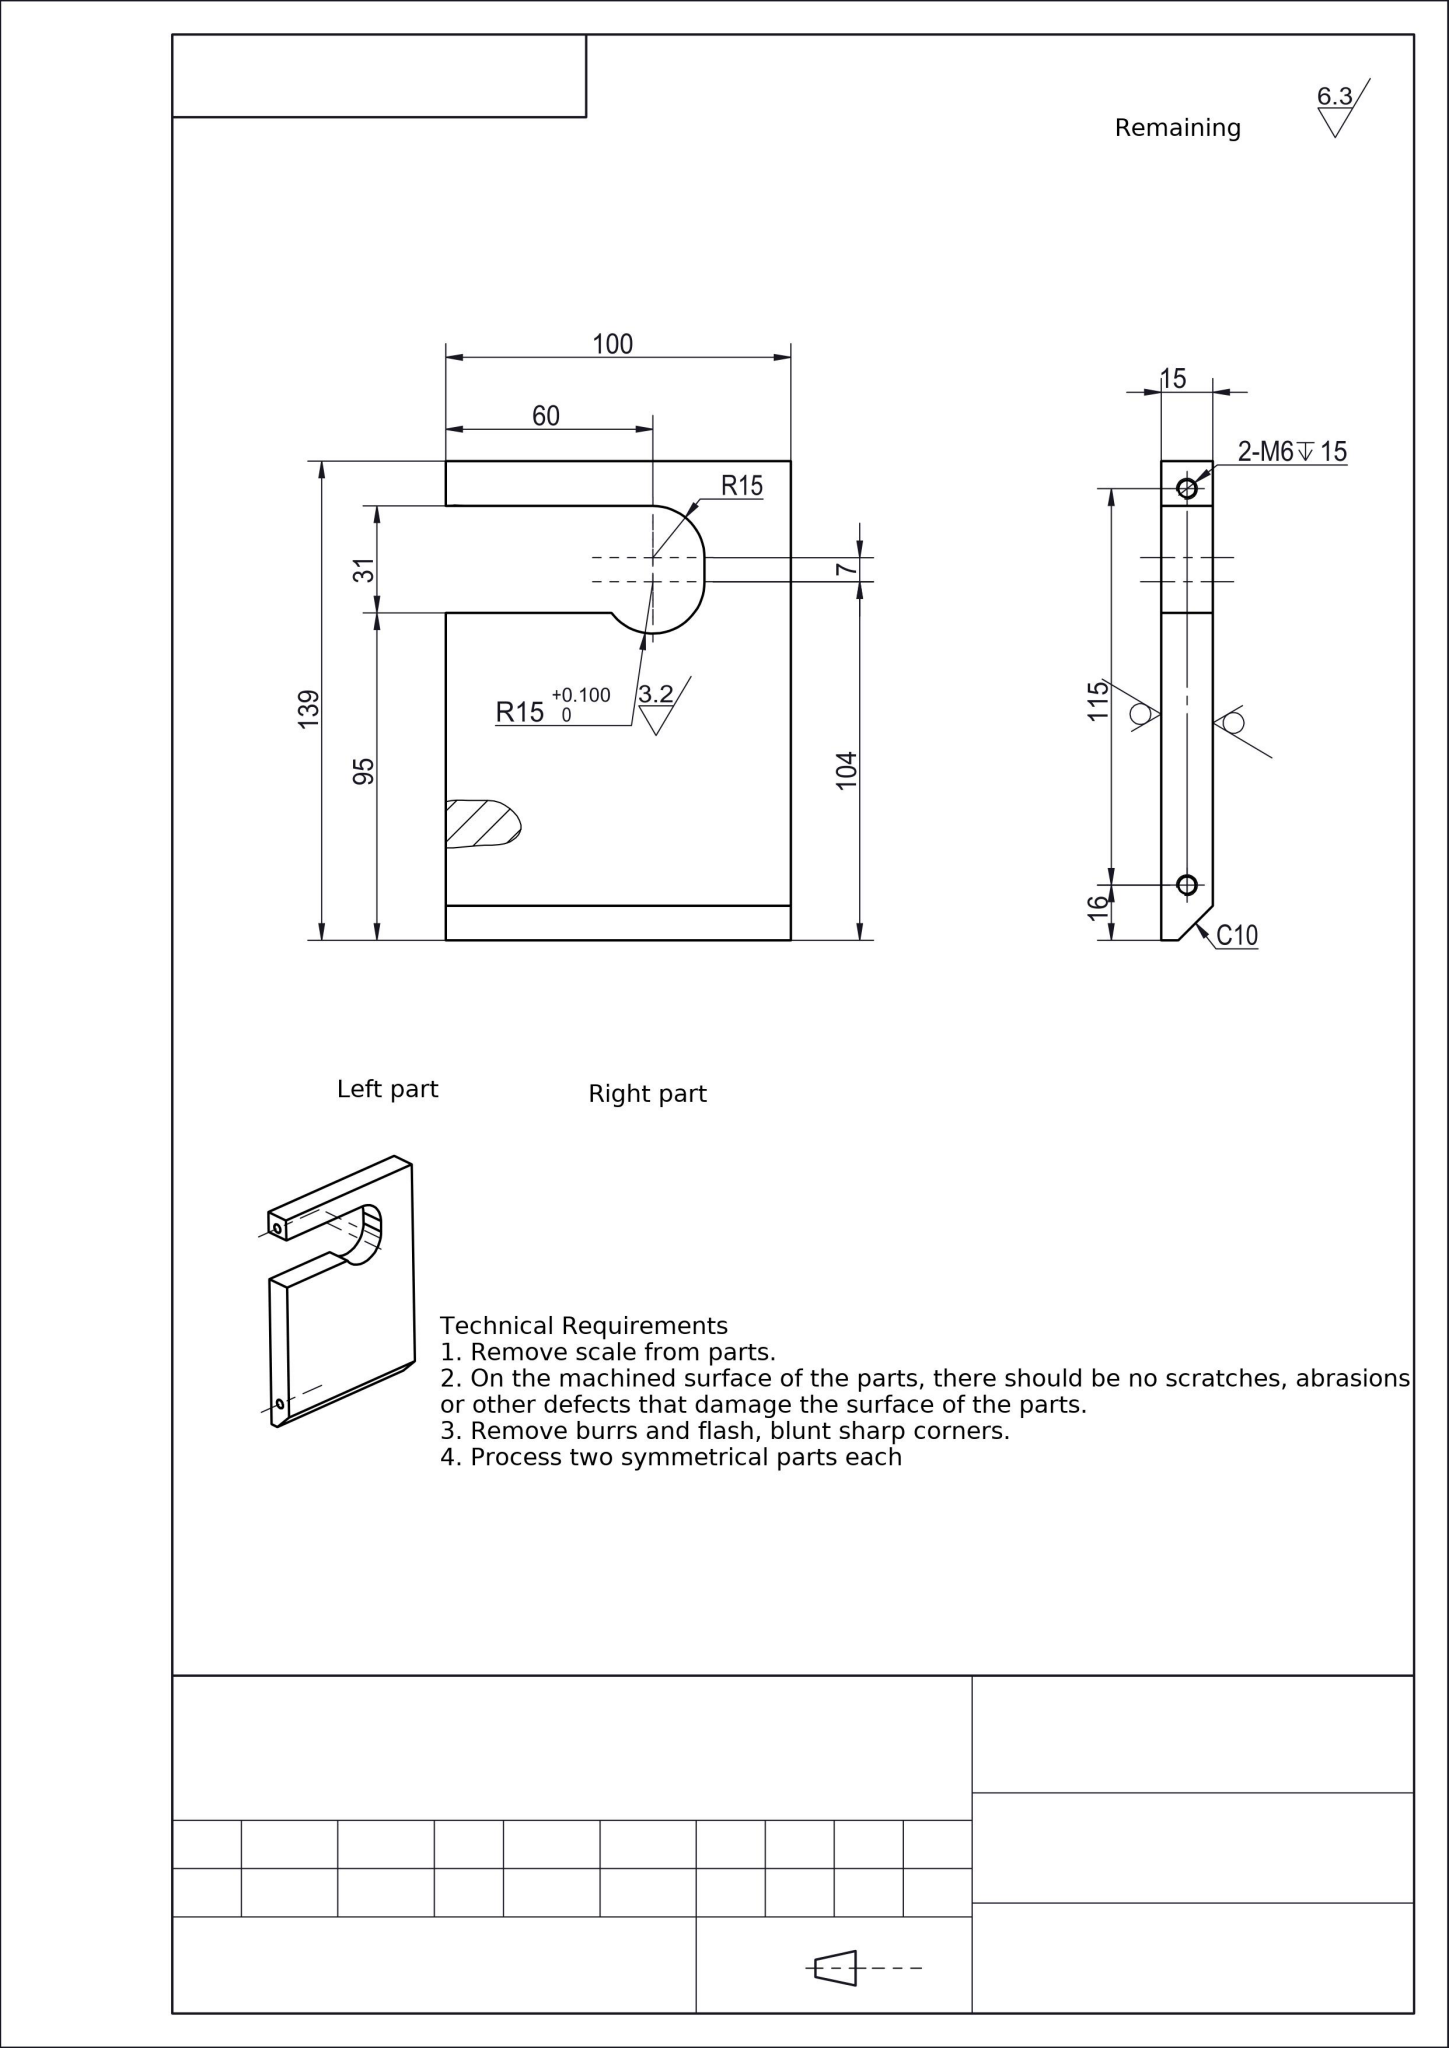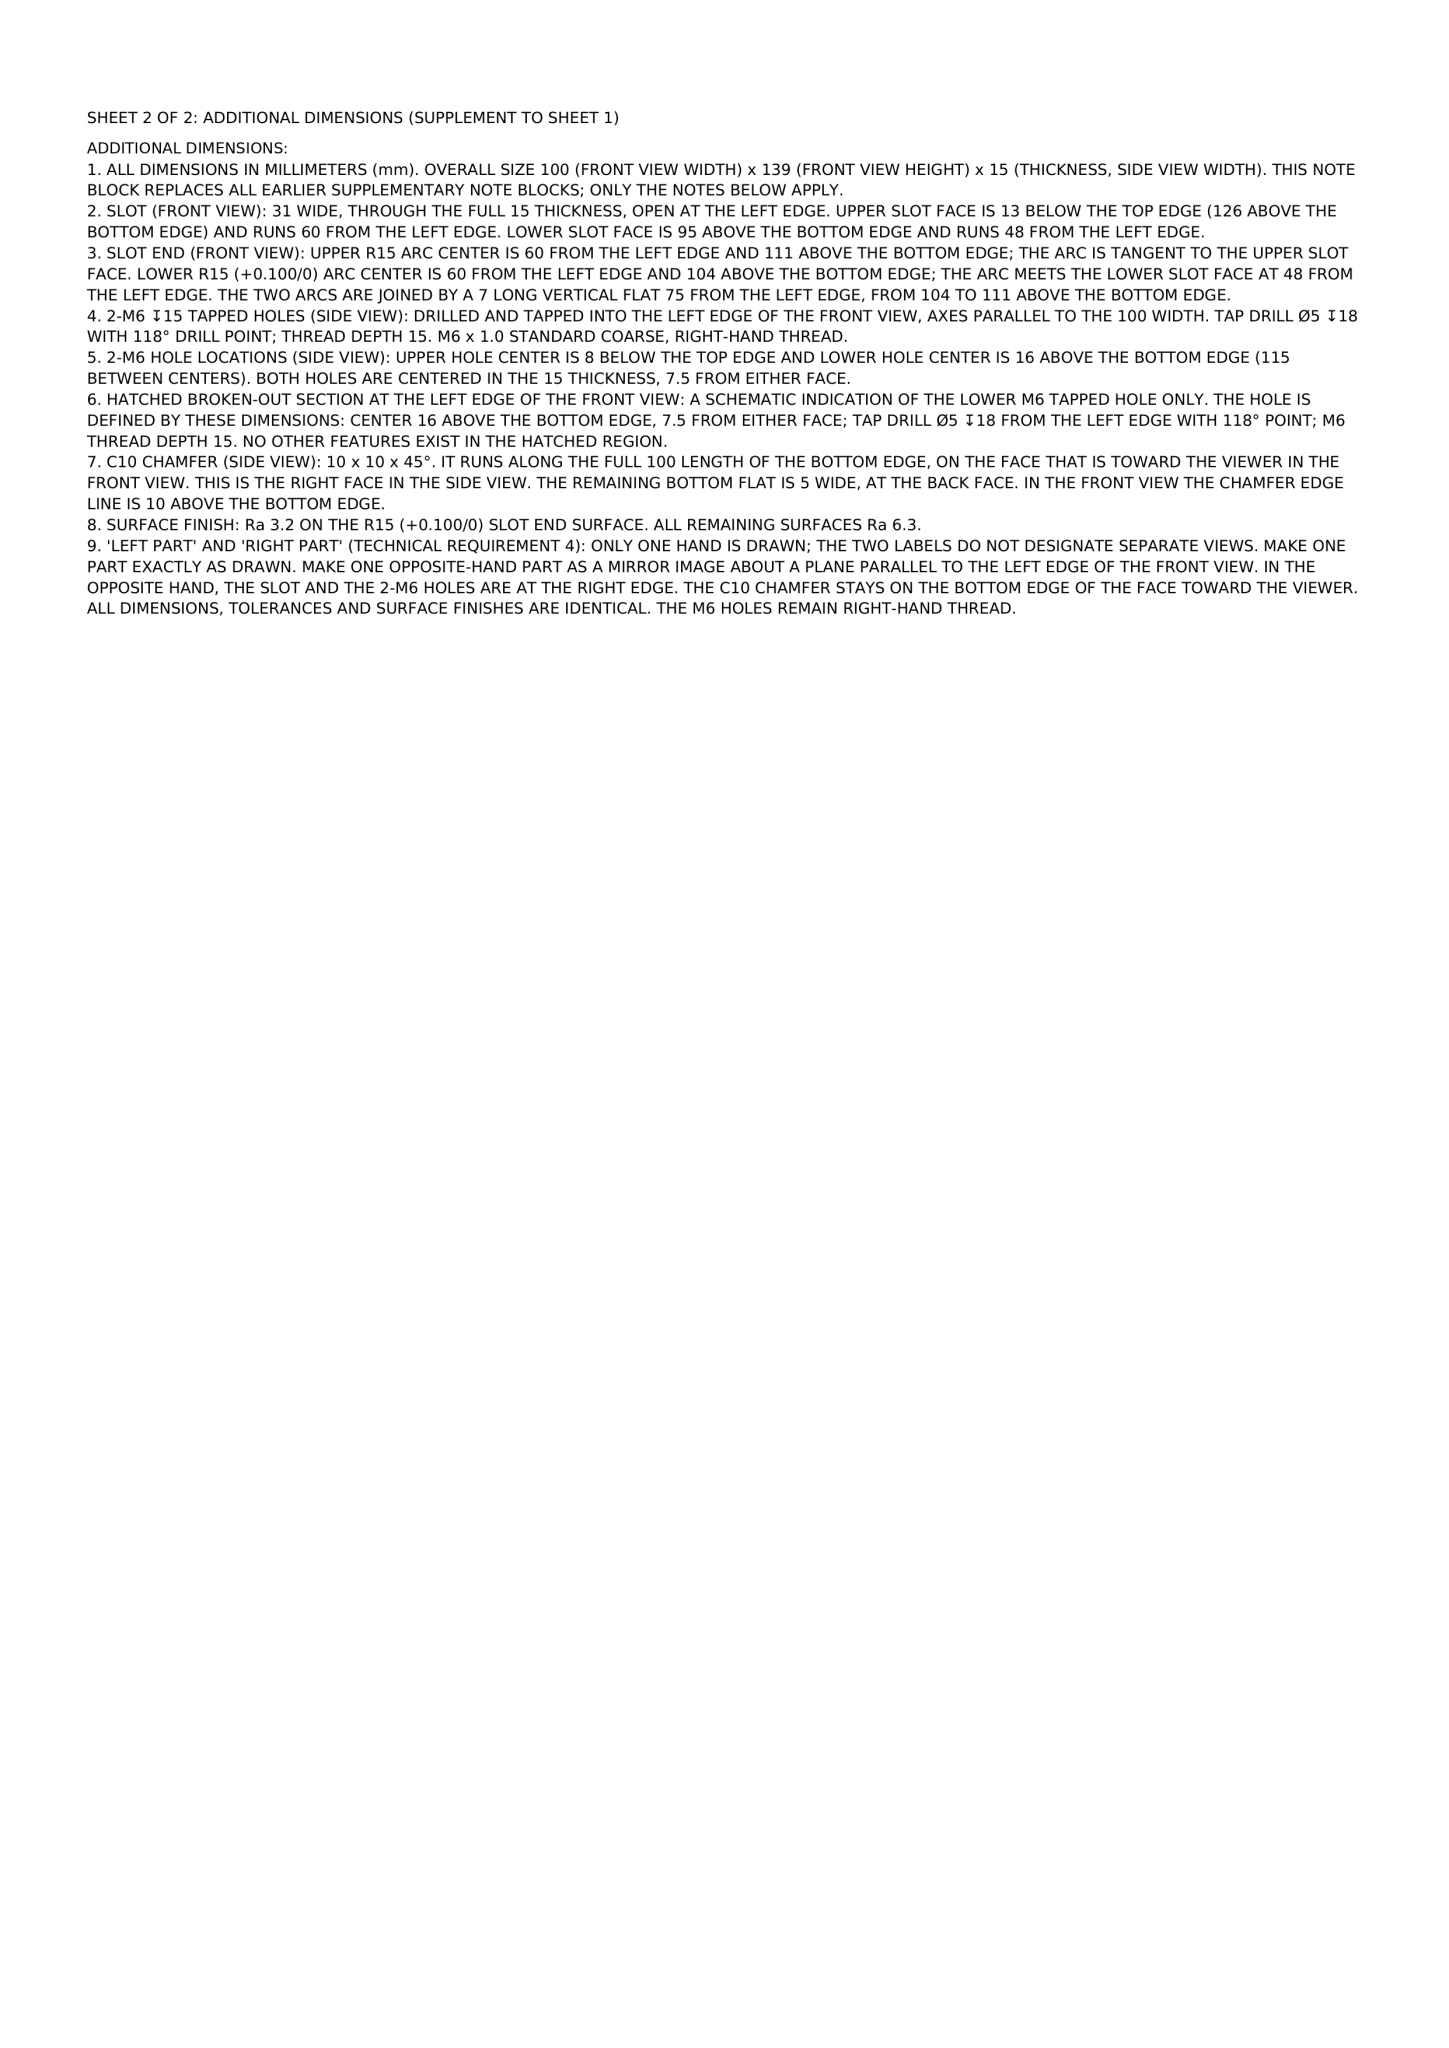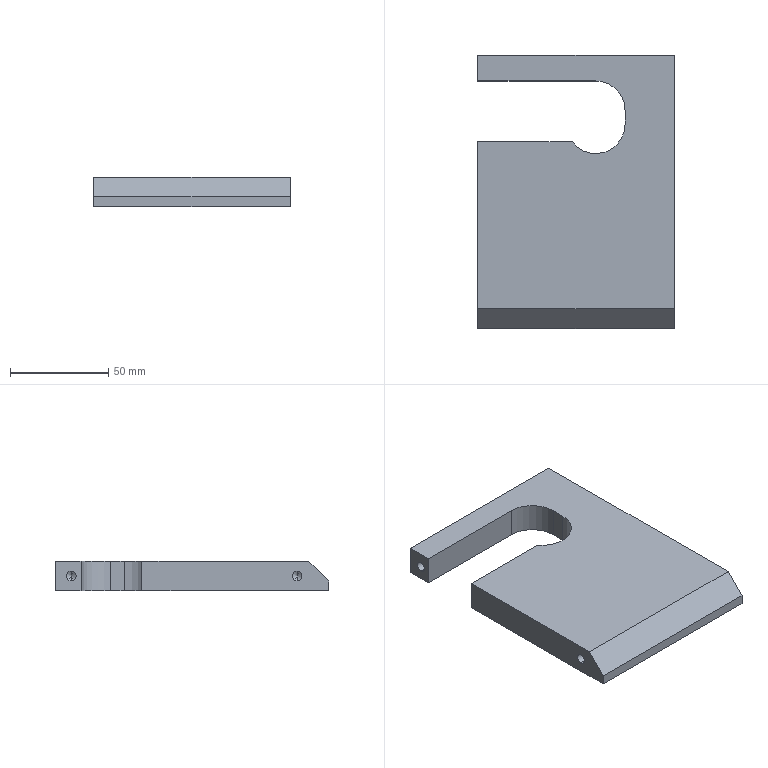Part | NX | mm | 1 solid | 21 faces | box 100 x 139 x 15 mm | volume 167242 mm3 | plane 11 | cylinder 6 | cone 4 | commonest cylinder face diameters 5 x4 30 x2
STEP:
#1=COLOUR_RGB('',0.7529,0.7529,0.7529);
#2=FILL_AREA_STYLE_COLOUR('',#1);
#3=FILL_AREA_STYLE('',(#2));
#4=SURFACE_STYLE_FILL_AREA(#3);
#5=SURFACE_SIDE_STYLE('',(#4));
#6=SURFACE_STYLE_USAGE(.BOTH.,#5);
#7=PRESENTATION_STYLE_ASSIGNMENT((#6));
#8=CARTESIAN_POINT('',(-32.,61.5,5.));
#9=VERTEX_POINT('',#8);
#10=CARTESIAN_POINT('',(-32.,61.5,10.));
#11=VERTEX_POINT('',#10);
#12=CARTESIAN_POINT('',(-32.,61.5,7.5));
#13=DIRECTION('',(-1.,-0.,0.));
#14=DIRECTION('',(0.,0.,1.));
#15=AXIS2_PLACEMENT_3D('',#12,#13,#14);
#16=CIRCLE('',#15,2.5);
#17=EDGE_CURVE('',#9,#11,#16,.T.);
#18=ORIENTED_EDGE('',*,*,#17,.F.);
#19=CARTESIAN_POINT('',(-50.,61.5,5.));
#20=VERTEX_POINT('',#19);
#21=CARTESIAN_POINT('',(-50.,61.5,5.));
#22=DIRECTION('',(-1.,-0.,0.));
#23=VECTOR('',#22,1000.);
#24=LINE('',#21,#23);
#25=EDGE_CURVE('',#9,#20,#24,.T.);
#26=ORIENTED_EDGE('',*,*,#25,.T.);
#27=CARTESIAN_POINT('',(-50.,61.5,10.));
#28=VERTEX_POINT('',#27);
#29=CARTESIAN_POINT('',(-50.,61.5,7.5));
#30=DIRECTION('',(-1.,-0.,0.));
#31=DIRECTION('',(0.,0.,1.));
#32=AXIS2_PLACEMENT_3D('',#29,#30,#31);
#33=CIRCLE('',#32,2.5);
#34=EDGE_CURVE('',#20,#28,#33,.T.);
#35=ORIENTED_EDGE('',*,*,#34,.T.);
#36=CARTESIAN_POINT('',(-50.,61.5,10.));
#37=DIRECTION('',(-1.,-0.,0.));
#38=VECTOR('',#37,1000.);
#39=LINE('',#36,#38);
#40=EDGE_CURVE('',#11,#28,#39,.T.);
#41=ORIENTED_EDGE('',*,*,#40,.F.);
#42=EDGE_LOOP('',(#18,#26,#35,#41));
#43=FACE_OUTER_BOUND('',#42,.T.);
#44=CARTESIAN_POINT('',(-50.,61.5,7.5));
#45=DIRECTION('',(-1.,-0.,0.));
#46=DIRECTION('',(0.,0.,1.));
#47=AXIS2_PLACEMENT_3D('',#44,#45,#46);
#48=CYLINDRICAL_SURFACE('',#47,2.5);
#49=ADVANCED_FACE('',(#43),#48,.F.);
#50=STYLED_ITEM('',(#7),#49);
#51=(LENGTH_UNIT()NAMED_UNIT(*)SI_UNIT(.MILLI.,.METRE.));
#52=UNCERTAINTY_MEASURE_WITH_UNIT(LENGTH_MEASURE(0.00001),#51,'','');
#53=(NAMED_UNIT(*)PLANE_ANGLE_UNIT()SI_UNIT($,.RADIAN.));
#54=(NAMED_UNIT(*)SI_UNIT($,.STERADIAN.)SOLID_ANGLE_UNIT());
#55=(GEOMETRIC_REPRESENTATION_CONTEXT(3)GLOBAL_UNCERTAINTY_ASSIGNED_CONTEXT((#52))GLOBAL_UNIT_ASSIGNED_CONTEXT((#51,#53,#54))REPRESENTATION_CONTEXT('',''));
#56=MECHANICAL_DESIGN_GEOMETRIC_PRESENTATION_REPRESENTATION('',(#50),#55);
#57=COLOUR_RGB('',1.,1.,1.);
#58=FILL_AREA_STYLE_COLOUR('',#57);
#59=FILL_AREA_STYLE('',(#58));
#60=SURFACE_STYLE_FILL_AREA(#59);
#61=SURFACE_SIDE_STYLE('',(#60));
#62=SURFACE_STYLE_USAGE(.BOTH.,#61);
#63=PRESENTATION_STYLE_ASSIGNMENT((#62));
#64=CARTESIAN_POINT('',(-30.498,61.5,7.5));
#65=VERTEX_POINT('',#64);
#66=CARTESIAN_POINT('',(-32.,61.5,10.));
#67=DIRECTION('',(-0.515,-0.,0.8572));
#68=VECTOR('',#67,1000.);
#69=LINE('',#66,#68);
#70=EDGE_CURVE('',#65,#11,#69,.T.);
#71=ORIENTED_EDGE('',*,*,#70,.F.);
#72=CARTESIAN_POINT('',(-32.,61.5,5.));
#73=DIRECTION('',(-0.515,0.,-0.8572));
#74=VECTOR('',#73,1000.);
#75=LINE('',#72,#74);
#76=EDGE_CURVE('',#65,#9,#75,.T.);
#77=ORIENTED_EDGE('',*,*,#76,.T.);
#78=ORIENTED_EDGE('',*,*,#17,.T.);
#79=EDGE_LOOP('',(#71,#77,#78));
#80=FACE_OUTER_BOUND('',#79,.T.);
#81=CARTESIAN_POINT('',(-32.,61.5,7.5));
#82=DIRECTION('',(-1.,-0.,0.));
#83=DIRECTION('',(0.,0.,1.));
#84=AXIS2_PLACEMENT_3D('',#81,#82,#83);
#85=CONICAL_SURFACE('',#84,2.5,1.03);
#86=ADVANCED_FACE('',(#80),#85,.F.);
#87=CARTESIAN_POINT('',(-32.,-53.5,5.));
#88=VERTEX_POINT('',#87);
#89=CARTESIAN_POINT('',(-32.,-53.5,10.));
#90=VERTEX_POINT('',#89);
#91=CARTESIAN_POINT('',(-32.,-53.5,7.5));
#92=DIRECTION('',(-1.,-0.,0.));
#93=DIRECTION('',(0.,0.,1.));
#94=AXIS2_PLACEMENT_3D('',#91,#92,#93);
#95=CIRCLE('',#94,2.5);
#96=EDGE_CURVE('',#88,#90,#95,.T.);
#97=ORIENTED_EDGE('',*,*,#96,.F.);
#98=CARTESIAN_POINT('',(-50.,-53.5,5.));
#99=VERTEX_POINT('',#98);
#100=CARTESIAN_POINT('',(-50.,-53.5,5.));
#101=DIRECTION('',(-1.,-0.,0.));
#102=VECTOR('',#101,1000.);
#103=LINE('',#100,#102);
#104=EDGE_CURVE('',#88,#99,#103,.T.);
#105=ORIENTED_EDGE('',*,*,#104,.T.);
#106=CARTESIAN_POINT('',(-50.,-53.5,10.));
#107=VERTEX_POINT('',#106);
#108=CARTESIAN_POINT('',(-50.,-53.5,7.5));
#109=DIRECTION('',(-1.,-0.,0.));
#110=DIRECTION('',(0.,0.,1.));
#111=AXIS2_PLACEMENT_3D('',#108,#109,#110);
#112=CIRCLE('',#111,2.5);
#113=EDGE_CURVE('',#99,#107,#112,.T.);
#114=ORIENTED_EDGE('',*,*,#113,.T.);
#115=CARTESIAN_POINT('',(-50.,-53.5,10.));
#116=DIRECTION('',(-1.,-0.,0.));
#117=VECTOR('',#116,1000.);
#118=LINE('',#115,#117);
#119=EDGE_CURVE('',#90,#107,#118,.T.);
#120=ORIENTED_EDGE('',*,*,#119,.F.);
#121=EDGE_LOOP('',(#97,#105,#114,#120));
#122=FACE_OUTER_BOUND('',#121,.T.);
#123=CARTESIAN_POINT('',(-50.,-53.5,7.5));
#124=DIRECTION('',(-1.,-0.,0.));
#125=DIRECTION('',(0.,0.,1.));
#126=AXIS2_PLACEMENT_3D('',#123,#124,#125);
#127=CYLINDRICAL_SURFACE('',#126,2.5);
#128=ADVANCED_FACE('',(#122),#127,.F.);
#129=CARTESIAN_POINT('',(-30.498,-53.5,7.5));
#130=VERTEX_POINT('',#129);
#131=CARTESIAN_POINT('',(-32.,-53.5,10.));
#132=DIRECTION('',(-0.515,-0.,0.8572));
#133=VECTOR('',#132,1000.);
#134=LINE('',#131,#133);
#135=EDGE_CURVE('',#130,#90,#134,.T.);
#136=ORIENTED_EDGE('',*,*,#135,.F.);
#137=CARTESIAN_POINT('',(-32.,-53.5,5.));
#138=DIRECTION('',(-0.515,0.,-0.8572));
#139=VECTOR('',#138,1000.);
#140=LINE('',#137,#139);
#141=EDGE_CURVE('',#130,#88,#140,.T.);
#142=ORIENTED_EDGE('',*,*,#141,.T.);
#143=ORIENTED_EDGE('',*,*,#96,.T.);
#144=EDGE_LOOP('',(#136,#142,#143));
#145=FACE_OUTER_BOUND('',#144,.T.);
#146=CARTESIAN_POINT('',(-32.,-53.5,7.5));
#147=DIRECTION('',(-1.,-0.,0.));
#148=DIRECTION('',(0.,0.,1.));
#149=AXIS2_PLACEMENT_3D('',#146,#147,#148);
#150=CONICAL_SURFACE('',#149,2.5,1.03);
#151=ADVANCED_FACE('',(#145),#150,.F.);
#152=CARTESIAN_POINT('',(-50.,25.5,15.));
#153=VERTEX_POINT('',#152);
#154=CARTESIAN_POINT('',(-50.,-59.5,15.));
#155=VERTEX_POINT('',#154);
#156=CARTESIAN_POINT('',(-50.,69.5,15.));
#157=DIRECTION('',(0.,-1.,0.));
#158=VECTOR('',#157,1000.);
#159=LINE('',#156,#158);
#160=EDGE_CURVE('',#153,#155,#159,.T.);
#161=ORIENTED_EDGE('',*,*,#160,.T.);
#162=CARTESIAN_POINT('',(50.,-59.5,15.));
#163=VERTEX_POINT('',#162);
#164=CARTESIAN_POINT('',(50.,-59.5,15.));
#165=DIRECTION('',(1.,0.,-0.));
#166=VECTOR('',#165,1000.);
#167=LINE('',#164,#166);
#168=EDGE_CURVE('',#155,#163,#167,.T.);
#169=ORIENTED_EDGE('',*,*,#168,.T.);
#170=CARTESIAN_POINT('',(50.,69.5,15.));
#171=VERTEX_POINT('',#170);
#172=CARTESIAN_POINT('',(50.,69.5,15.));
#173=DIRECTION('',(0.,1.,-0.));
#174=VECTOR('',#173,1000.);
#175=LINE('',#172,#174);
#176=EDGE_CURVE('',#163,#171,#175,.T.);
#177=ORIENTED_EDGE('',*,*,#176,.T.);
#178=CARTESIAN_POINT('',(-50.,69.5,15.));
#179=VERTEX_POINT('',#178);
#180=CARTESIAN_POINT('',(-50.,69.5,15.));
#181=DIRECTION('',(-1.,-0.,0.));
#182=VECTOR('',#181,1000.);
#183=LINE('',#180,#182);
#184=EDGE_CURVE('',#171,#179,#183,.T.);
#185=ORIENTED_EDGE('',*,*,#184,.T.);
#186=CARTESIAN_POINT('',(-50.,56.5,15.));
#187=VERTEX_POINT('',#186);
#188=CARTESIAN_POINT('',(-50.,69.5,15.));
#189=DIRECTION('',(0.,-1.,0.));
#190=VECTOR('',#189,1000.);
#191=LINE('',#188,#190);
#192=EDGE_CURVE('',#179,#187,#191,.T.);
#193=ORIENTED_EDGE('',*,*,#192,.T.);
#194=CARTESIAN_POINT('',(10.,56.5,15.));
#195=VERTEX_POINT('',#194);
#196=CARTESIAN_POINT('',(-112.137,56.5,15.));
#197=DIRECTION('',(-1.,-0.,0.));
#198=VECTOR('',#197,1000.);
#199=LINE('',#196,#198);
#200=EDGE_CURVE('',#195,#187,#199,.T.);
#201=ORIENTED_EDGE('',*,*,#200,.F.);
#202=CARTESIAN_POINT('',(25.,41.5,15.));
#203=VERTEX_POINT('',#202);
#204=CARTESIAN_POINT('',(10.,41.5,15.));
#205=DIRECTION('',(-0.,-0.,1.));
#206=DIRECTION('',(1.,0.,-0.));
#207=AXIS2_PLACEMENT_3D('',#204,#205,#206);
#208=CIRCLE('',#207,15.);
#209=EDGE_CURVE('',#203,#195,#208,.T.);
#210=ORIENTED_EDGE('',*,*,#209,.F.);
#211=CARTESIAN_POINT('',(25.,34.5,15.));
#212=VERTEX_POINT('',#211);
#213=CARTESIAN_POINT('',(25.,41.5,15.));
#214=DIRECTION('',(0.,1.,-0.));
#215=VECTOR('',#214,1000.);
#216=LINE('',#213,#215);
#217=EDGE_CURVE('',#212,#203,#216,.T.);
#218=ORIENTED_EDGE('',*,*,#217,.F.);
#219=CARTESIAN_POINT('',(-2.,25.5,15.));
#220=VERTEX_POINT('',#219);
#221=CARTESIAN_POINT('',(10.,34.5,15.));
#222=DIRECTION('',(-0.,-0.,1.));
#223=DIRECTION('',(1.,0.,-0.));
#224=AXIS2_PLACEMENT_3D('',#221,#222,#223);
#225=CIRCLE('',#224,15.);
#226=EDGE_CURVE('',#220,#212,#225,.T.);
#227=ORIENTED_EDGE('',*,*,#226,.F.);
#228=CARTESIAN_POINT('',(-112.137,25.5,15.));
#229=DIRECTION('',(1.,0.,-0.));
#230=VECTOR('',#229,1000.);
#231=LINE('',#228,#230);
#232=EDGE_CURVE('',#153,#220,#231,.T.);
#233=ORIENTED_EDGE('',*,*,#232,.F.);
#234=EDGE_LOOP('',(#161,#169,#177,#185,#193,#201,#210,#218,#227,#233));
#235=FACE_OUTER_BOUND('',#234,.T.);
#236=CARTESIAN_POINT('',(0.,0.,15.));
#237=DIRECTION('',(0.,-0.,1.));
#238=DIRECTION('',(1.,0.,-0.));
#239=AXIS2_PLACEMENT_3D('',#236,#237,#238);
#240=PLANE('',#239);
#241=ADVANCED_FACE('',(#235),#240,.T.);
#242=CARTESIAN_POINT('',(25.,41.5,-0.));
#243=VERTEX_POINT('',#242);
#244=CARTESIAN_POINT('',(10.,56.5,-0.));
#245=VERTEX_POINT('',#244);
#246=CARTESIAN_POINT('',(10.,41.5,-0.));
#247=DIRECTION('',(-0.,-0.,1.));
#248=DIRECTION('',(1.,0.,-0.));
#249=AXIS2_PLACEMENT_3D('',#246,#247,#248);
#250=CIRCLE('',#249,15.);
#251=EDGE_CURVE('',#243,#245,#250,.T.);
#252=ORIENTED_EDGE('',*,*,#251,.T.);
#253=CARTESIAN_POINT('',(-50.,56.5,-0.));
#254=VERTEX_POINT('',#253);
#255=CARTESIAN_POINT('',(-112.137,56.5,-0.));
#256=DIRECTION('',(-1.,-0.,0.));
#257=VECTOR('',#256,1000.);
#258=LINE('',#255,#257);
#259=EDGE_CURVE('',#245,#254,#258,.T.);
#260=ORIENTED_EDGE('',*,*,#259,.T.);
#261=CARTESIAN_POINT('',(-50.,69.5,-0.));
#262=VERTEX_POINT('',#261);
#263=CARTESIAN_POINT('',(-50.,69.5,-0.));
#264=DIRECTION('',(0.,-1.,0.));
#265=VECTOR('',#264,1000.);
#266=LINE('',#263,#265);
#267=EDGE_CURVE('',#262,#254,#266,.T.);
#268=ORIENTED_EDGE('',*,*,#267,.F.);
#269=CARTESIAN_POINT('',(50.,69.5,-0.));
#270=VERTEX_POINT('',#269);
#271=CARTESIAN_POINT('',(-50.,69.5,-0.));
#272=DIRECTION('',(-1.,-0.,0.));
#273=VECTOR('',#272,1000.);
#274=LINE('',#271,#273);
#275=EDGE_CURVE('',#270,#262,#274,.T.);
#276=ORIENTED_EDGE('',*,*,#275,.F.);
#277=CARTESIAN_POINT('',(50.,-69.5,0.));
#278=VERTEX_POINT('',#277);
#279=CARTESIAN_POINT('',(50.,69.5,-0.));
#280=DIRECTION('',(0.,1.,-0.));
#281=VECTOR('',#280,1000.);
#282=LINE('',#279,#281);
#283=EDGE_CURVE('',#278,#270,#282,.T.);
#284=ORIENTED_EDGE('',*,*,#283,.F.);
#285=CARTESIAN_POINT('',(-50.,-69.5,0.));
#286=VERTEX_POINT('',#285);
#287=CARTESIAN_POINT('',(-50.,-69.5,0.));
#288=DIRECTION('',(1.,0.,-0.));
#289=VECTOR('',#288,1000.);
#290=LINE('',#287,#289);
#291=EDGE_CURVE('',#286,#278,#290,.T.);
#292=ORIENTED_EDGE('',*,*,#291,.F.);
#293=CARTESIAN_POINT('',(-50.,25.5,-0.));
#294=VERTEX_POINT('',#293);
#295=CARTESIAN_POINT('',(-50.,69.5,-0.));
#296=DIRECTION('',(0.,-1.,0.));
#297=VECTOR('',#296,1000.);
#298=LINE('',#295,#297);
#299=EDGE_CURVE('',#294,#286,#298,.T.);
#300=ORIENTED_EDGE('',*,*,#299,.F.);
#301=CARTESIAN_POINT('',(-2.,25.5,-0.));
#302=VERTEX_POINT('',#301);
#303=CARTESIAN_POINT('',(0.,25.5,-0.));
#304=DIRECTION('',(-1.,-0.,0.));
#305=VECTOR('',#304,1000.);
#306=LINE('',#303,#305);
#307=EDGE_CURVE('',#302,#294,#306,.T.);
#308=ORIENTED_EDGE('',*,*,#307,.F.);
#309=CARTESIAN_POINT('',(25.,34.5,-0.));
#310=VERTEX_POINT('',#309);
#311=CARTESIAN_POINT('',(10.,34.5,-0.));
#312=DIRECTION('',(-0.,-0.,1.));
#313=DIRECTION('',(1.,0.,-0.));
#314=AXIS2_PLACEMENT_3D('',#311,#312,#313);
#315=CIRCLE('',#314,15.);
#316=EDGE_CURVE('',#302,#310,#315,.T.);
#317=ORIENTED_EDGE('',*,*,#316,.T.);
#318=CARTESIAN_POINT('',(25.,41.5,-0.));
#319=DIRECTION('',(0.,1.,-0.));
#320=VECTOR('',#319,1000.);
#321=LINE('',#318,#320);
#322=EDGE_CURVE('',#310,#243,#321,.T.);
#323=ORIENTED_EDGE('',*,*,#322,.T.);
#324=EDGE_LOOP('',(#252,#260,#268,#276,#284,#292,#300,#308,#317,#323));
#325=FACE_OUTER_BOUND('',#324,.T.);
#326=CARTESIAN_POINT('',(0.,0.,0.));
#327=DIRECTION('',(0.,-0.,1.));
#328=DIRECTION('',(1.,0.,-0.));
#329=AXIS2_PLACEMENT_3D('',#326,#327,#328);
#330=PLANE('',#329);
#331=ADVANCED_FACE('',(#325),#330,.F.);
#332=ORIENTED_EDGE('',*,*,#232,.T.);
#333=CARTESIAN_POINT('',(-2.,25.5,15.));
#334=DIRECTION('',(0.,0.,-1.));
#335=VECTOR('',#334,1000.);
#336=LINE('',#333,#335);
#337=EDGE_CURVE('',#220,#302,#336,.T.);
#338=ORIENTED_EDGE('',*,*,#337,.T.);
#339=ORIENTED_EDGE('',*,*,#307,.T.);
#340=CARTESIAN_POINT('',(-50.,25.5,15.));
#341=DIRECTION('',(-0.,-0.,1.));
#342=VECTOR('',#341,1000.);
#343=LINE('',#340,#342);
#344=EDGE_CURVE('',#294,#153,#343,.T.);
#345=ORIENTED_EDGE('',*,*,#344,.T.);
#346=EDGE_LOOP('',(#332,#338,#339,#345));
#347=FACE_OUTER_BOUND('',#346,.T.);
#348=CARTESIAN_POINT('',(-112.137,25.5,15.));
#349=DIRECTION('',(0.,1.,0.));
#350=DIRECTION('',(-0.,-0.,1.));
#351=AXIS2_PLACEMENT_3D('',#348,#349,#350);
#352=PLANE('',#351);
#353=ADVANCED_FACE('',(#347),#352,.T.);
#354=CARTESIAN_POINT('',(-50.,61.5,7.5));
#355=DIRECTION('',(-1.,-0.,0.));
#356=DIRECTION('',(0.,0.,1.));
#357=AXIS2_PLACEMENT_3D('',#354,#355,#356);
#358=CIRCLE('',#357,2.5);
#359=EDGE_CURVE('',#28,#20,#358,.T.);
#360=ORIENTED_EDGE('',*,*,#359,.F.);
#361=ORIENTED_EDGE('',*,*,#34,.F.);
#362=EDGE_LOOP('',(#360,#361));
#363=FACE_BOUND('',#362,.T.);
#364=CARTESIAN_POINT('',(-50.,56.5,15.));
#365=DIRECTION('',(0.,0.,-1.));
#366=VECTOR('',#365,1000.);
#367=LINE('',#364,#366);
#368=EDGE_CURVE('',#187,#254,#367,.T.);
#369=ORIENTED_EDGE('',*,*,#368,.F.);
#370=ORIENTED_EDGE('',*,*,#192,.F.);
#371=CARTESIAN_POINT('',(-50.,69.5,15.));
#372=DIRECTION('',(0.,0.,-1.));
#373=VECTOR('',#372,1000.);
#374=LINE('',#371,#373);
#375=EDGE_CURVE('',#179,#262,#374,.T.);
#376=ORIENTED_EDGE('',*,*,#375,.T.);
#377=ORIENTED_EDGE('',*,*,#267,.T.);
#378=EDGE_LOOP('',(#369,#370,#376,#377));
#379=FACE_OUTER_BOUND('',#378,.T.);
#380=CARTESIAN_POINT('',(-50.,69.5,15.));
#381=DIRECTION('',(1.,0.,-0.));
#382=DIRECTION('',(-0.,1.,-0.));
#383=AXIS2_PLACEMENT_3D('',#380,#381,#382);
#384=PLANE('',#383);
#385=ADVANCED_FACE('',(#363,#379),#384,.F.);
#386=CARTESIAN_POINT('',(-50.,-53.5,7.5));
#387=DIRECTION('',(-1.,-0.,0.));
#388=DIRECTION('',(0.,0.,1.));
#389=AXIS2_PLACEMENT_3D('',#386,#387,#388);
#390=CIRCLE('',#389,2.5);
#391=EDGE_CURVE('',#107,#99,#390,.T.);
#392=ORIENTED_EDGE('',*,*,#391,.F.);
#393=ORIENTED_EDGE('',*,*,#113,.F.);
#394=EDGE_LOOP('',(#392,#393));
#395=FACE_BOUND('',#394,.T.);
#396=CARTESIAN_POINT('',(-50.,-69.5,5.));
#397=VERTEX_POINT('',#396);
#398=CARTESIAN_POINT('',(-50.,-69.5,15.));
#399=DIRECTION('',(0.,0.,-1.));
#400=VECTOR('',#399,1000.);
#401=LINE('',#398,#400);
#402=EDGE_CURVE('',#397,#286,#401,.T.);
#403=ORIENTED_EDGE('',*,*,#402,.F.);
#404=CARTESIAN_POINT('',(-50.,-59.5,15.));
#405=DIRECTION('',(-0.,0.7071,0.7071));
#406=VECTOR('',#405,1000.);
#407=LINE('',#404,#406);
#408=EDGE_CURVE('',#397,#155,#407,.T.);
#409=ORIENTED_EDGE('',*,*,#408,.T.);
#410=ORIENTED_EDGE('',*,*,#160,.F.);
#411=ORIENTED_EDGE('',*,*,#344,.F.);
#412=ORIENTED_EDGE('',*,*,#299,.T.);
#413=EDGE_LOOP('',(#403,#409,#410,#411,#412));
#414=FACE_OUTER_BOUND('',#413,.T.);
#415=CARTESIAN_POINT('',(-50.,69.5,15.));
#416=DIRECTION('',(1.,0.,-0.));
#417=DIRECTION('',(-0.,1.,-0.));
#418=AXIS2_PLACEMENT_3D('',#415,#416,#417);
#419=PLANE('',#418);
#420=ADVANCED_FACE('',(#395,#414),#419,.F.);
#421=ORIENTED_EDGE('',*,*,#176,.F.);
#422=CARTESIAN_POINT('',(50.,-69.5,5.));
#423=VERTEX_POINT('',#422);
#424=CARTESIAN_POINT('',(50.,-59.5,15.));
#425=DIRECTION('',(0.,-0.7071,-0.7071));
#426=VECTOR('',#425,1000.);
#427=LINE('',#424,#426);
#428=EDGE_CURVE('',#163,#423,#427,.T.);
#429=ORIENTED_EDGE('',*,*,#428,.T.);
#430=CARTESIAN_POINT('',(50.,-69.5,15.));
#431=DIRECTION('',(0.,0.,-1.));
#432=VECTOR('',#431,1000.);
#433=LINE('',#430,#432);
#434=EDGE_CURVE('',#423,#278,#433,.T.);
#435=ORIENTED_EDGE('',*,*,#434,.T.);
#436=ORIENTED_EDGE('',*,*,#283,.T.);
#437=CARTESIAN_POINT('',(50.,69.5,15.));
#438=DIRECTION('',(0.,0.,-1.));
#439=VECTOR('',#438,1000.);
#440=LINE('',#437,#439);
#441=EDGE_CURVE('',#171,#270,#440,.T.);
#442=ORIENTED_EDGE('',*,*,#441,.F.);
#443=EDGE_LOOP('',(#421,#429,#435,#436,#442));
#444=FACE_OUTER_BOUND('',#443,.T.);
#445=CARTESIAN_POINT('',(50.,69.5,15.));
#446=DIRECTION('',(-1.,0.,0.));
#447=DIRECTION('',(-0.,-1.,0.));
#448=AXIS2_PLACEMENT_3D('',#445,#446,#447);
#449=PLANE('',#448);
#450=ADVANCED_FACE('',(#444),#449,.F.);
#451=ORIENTED_EDGE('',*,*,#275,.T.);
#452=ORIENTED_EDGE('',*,*,#375,.F.);
#453=ORIENTED_EDGE('',*,*,#184,.F.);
#454=ORIENTED_EDGE('',*,*,#441,.T.);
#455=EDGE_LOOP('',(#451,#452,#453,#454));
#456=FACE_OUTER_BOUND('',#455,.T.);
#457=CARTESIAN_POINT('',(-50.,69.5,15.));
#458=DIRECTION('',(-0.,-1.,-0.));
#459=DIRECTION('',(0.,0.,-1.));
#460=AXIS2_PLACEMENT_3D('',#457,#458,#459);
#461=PLANE('',#460);
#462=ADVANCED_FACE('',(#456),#461,.F.);
#463=ORIENTED_EDGE('',*,*,#434,.F.);
#464=CARTESIAN_POINT('',(-50.,-69.5,5.));
#465=DIRECTION('',(-1.,-0.,0.));
#466=VECTOR('',#465,1000.);
#467=LINE('',#464,#466);
#468=EDGE_CURVE('',#423,#397,#467,.T.);
#469=ORIENTED_EDGE('',*,*,#468,.T.);
#470=ORIENTED_EDGE('',*,*,#402,.T.);
#471=ORIENTED_EDGE('',*,*,#291,.T.);
#472=EDGE_LOOP('',(#463,#469,#470,#471));
#473=FACE_OUTER_BOUND('',#472,.T.);
#474=CARTESIAN_POINT('',(-50.,-69.5,15.));
#475=DIRECTION('',(0.,1.,0.));
#476=DIRECTION('',(-0.,-0.,1.));
#477=AXIS2_PLACEMENT_3D('',#474,#475,#476);
#478=PLANE('',#477);
#479=ADVANCED_FACE('',(#473),#478,.F.);
#480=ORIENTED_EDGE('',*,*,#368,.T.);
#481=ORIENTED_EDGE('',*,*,#259,.F.);
#482=CARTESIAN_POINT('',(10.,56.5,15.));
#483=DIRECTION('',(0.,0.,-1.));
#484=VECTOR('',#483,1000.);
#485=LINE('',#482,#484);
#486=EDGE_CURVE('',#195,#245,#485,.T.);
#487=ORIENTED_EDGE('',*,*,#486,.F.);
#488=ORIENTED_EDGE('',*,*,#200,.T.);
#489=EDGE_LOOP('',(#480,#481,#487,#488));
#490=FACE_OUTER_BOUND('',#489,.T.);
#491=CARTESIAN_POINT('',(-112.137,56.5,15.));
#492=DIRECTION('',(-0.,-1.,-0.));
#493=DIRECTION('',(0.,0.,-1.));
#494=AXIS2_PLACEMENT_3D('',#491,#492,#493);
#495=PLANE('',#494);
#496=ADVANCED_FACE('',(#490),#495,.T.);
#497=ORIENTED_EDGE('',*,*,#251,.F.);
#498=CARTESIAN_POINT('',(25.,41.5,15.));
#499=DIRECTION('',(0.,0.,-1.));
#500=VECTOR('',#499,1000.);
#501=LINE('',#498,#500);
#502=EDGE_CURVE('',#203,#243,#501,.T.);
#503=ORIENTED_EDGE('',*,*,#502,.F.);
#504=ORIENTED_EDGE('',*,*,#209,.T.);
#505=ORIENTED_EDGE('',*,*,#486,.T.);
#506=EDGE_LOOP('',(#497,#503,#504,#505));
#507=FACE_OUTER_BOUND('',#506,.T.);
#508=CARTESIAN_POINT('',(10.,41.5,15.));
#509=DIRECTION('',(0.,0.,-1.));
#510=DIRECTION('',(-1.,0.,0.));
#511=AXIS2_PLACEMENT_3D('',#508,#509,#510);
#512=CYLINDRICAL_SURFACE('',#511,15.);
#513=ADVANCED_FACE('',(#507),#512,.F.);
#514=ORIENTED_EDGE('',*,*,#226,.T.);
#515=CARTESIAN_POINT('',(25.,34.5,15.));
#516=DIRECTION('',(0.,0.,-1.));
#517=VECTOR('',#516,1000.);
#518=LINE('',#515,#517);
#519=EDGE_CURVE('',#212,#310,#518,.T.);
#520=ORIENTED_EDGE('',*,*,#519,.T.);
#521=ORIENTED_EDGE('',*,*,#316,.F.);
#522=ORIENTED_EDGE('',*,*,#337,.F.);
#523=EDGE_LOOP('',(#514,#520,#521,#522));
#524=FACE_OUTER_BOUND('',#523,.T.);
#525=CARTESIAN_POINT('',(10.,34.5,15.));
#526=DIRECTION('',(0.,0.,-1.));
#527=DIRECTION('',(-1.,0.,0.));
#528=AXIS2_PLACEMENT_3D('',#525,#526,#527);
#529=CYLINDRICAL_SURFACE('',#528,15.);
#530=ADVANCED_FACE('',(#524),#529,.F.);
#531=ORIENTED_EDGE('',*,*,#322,.F.);
#532=ORIENTED_EDGE('',*,*,#519,.F.);
#533=ORIENTED_EDGE('',*,*,#217,.T.);
#534=ORIENTED_EDGE('',*,*,#502,.T.);
#535=EDGE_LOOP('',(#531,#532,#533,#534));
#536=FACE_OUTER_BOUND('',#535,.T.);
#537=CARTESIAN_POINT('',(25.,41.5,15.));
#538=DIRECTION('',(-1.,0.,0.));
#539=DIRECTION('',(-0.,-1.,0.));
#540=AXIS2_PLACEMENT_3D('',#537,#538,#539);
#541=PLANE('',#540);
#542=ADVANCED_FACE('',(#536),#541,.T.);
#543=ORIENTED_EDGE('',*,*,#408,.F.);
#544=ORIENTED_EDGE('',*,*,#468,.F.);
#545=ORIENTED_EDGE('',*,*,#428,.F.);
#546=ORIENTED_EDGE('',*,*,#168,.F.);
#547=EDGE_LOOP('',(#543,#544,#545,#546));
#548=FACE_OUTER_BOUND('',#547,.T.);
#549=CARTESIAN_POINT('',(0.,-59.5,15.));
#550=DIRECTION('',(0.,-0.7071,0.7071));
#551=DIRECTION('',(-1.,-0.,0.));
#552=AXIS2_PLACEMENT_3D('',#549,#550,#551);
#553=PLANE('',#552);
#554=ADVANCED_FACE('',(#548),#553,.T.);
#555=ORIENTED_EDGE('',*,*,#141,.F.);
#556=ORIENTED_EDGE('',*,*,#135,.T.);
#557=CARTESIAN_POINT('',(-32.,-53.5,7.5));
#558=DIRECTION('',(-1.,-0.,0.));
#559=DIRECTION('',(0.,0.,1.));
#560=AXIS2_PLACEMENT_3D('',#557,#558,#559);
#561=CIRCLE('',#560,2.5);
#562=EDGE_CURVE('',#90,#88,#561,.T.);
#563=ORIENTED_EDGE('',*,*,#562,.T.);
#564=EDGE_LOOP('',(#555,#556,#563));
#565=FACE_OUTER_BOUND('',#564,.T.);
#566=CARTESIAN_POINT('',(-32.,-53.5,7.5));
#567=DIRECTION('',(-1.,-0.,0.));
#568=DIRECTION('',(0.,0.,1.));
#569=AXIS2_PLACEMENT_3D('',#566,#567,#568);
#570=CONICAL_SURFACE('',#569,2.5,1.03);
#571=ADVANCED_FACE('',(#565),#570,.F.);
#572=ORIENTED_EDGE('',*,*,#104,.F.);
#573=ORIENTED_EDGE('',*,*,#562,.F.);
#574=ORIENTED_EDGE('',*,*,#119,.T.);
#575=ORIENTED_EDGE('',*,*,#391,.T.);
#576=EDGE_LOOP('',(#572,#573,#574,#575));
#577=FACE_OUTER_BOUND('',#576,.T.);
#578=CARTESIAN_POINT('',(-50.,-53.5,7.5));
#579=DIRECTION('',(-1.,-0.,0.));
#580=DIRECTION('',(0.,0.,1.));
#581=AXIS2_PLACEMENT_3D('',#578,#579,#580);
#582=CYLINDRICAL_SURFACE('',#581,2.5);
#583=ADVANCED_FACE('',(#577),#582,.F.);
#584=ORIENTED_EDGE('',*,*,#76,.F.);
#585=ORIENTED_EDGE('',*,*,#70,.T.);
#586=CARTESIAN_POINT('',(-32.,61.5,7.5));
#587=DIRECTION('',(-1.,-0.,0.));
#588=DIRECTION('',(0.,0.,1.));
#589=AXIS2_PLACEMENT_3D('',#586,#587,#588);
#590=CIRCLE('',#589,2.5);
#591=EDGE_CURVE('',#11,#9,#590,.T.);
#592=ORIENTED_EDGE('',*,*,#591,.T.);
#593=EDGE_LOOP('',(#584,#585,#592));
#594=FACE_OUTER_BOUND('',#593,.T.);
#595=CARTESIAN_POINT('',(-32.,61.5,7.5));
#596=DIRECTION('',(-1.,-0.,0.));
#597=DIRECTION('',(0.,0.,1.));
#598=AXIS2_PLACEMENT_3D('',#595,#596,#597);
#599=CONICAL_SURFACE('',#598,2.5,1.03);
#600=ADVANCED_FACE('',(#594),#599,.F.);
#601=ORIENTED_EDGE('',*,*,#25,.F.);
#602=ORIENTED_EDGE('',*,*,#591,.F.);
#603=ORIENTED_EDGE('',*,*,#40,.T.);
#604=ORIENTED_EDGE('',*,*,#359,.T.);
#605=EDGE_LOOP('',(#601,#602,#603,#604));
#606=FACE_OUTER_BOUND('',#605,.T.);
#607=CARTESIAN_POINT('',(-50.,61.5,7.5));
#608=DIRECTION('',(-1.,-0.,0.));
#609=DIRECTION('',(0.,0.,1.));
#610=AXIS2_PLACEMENT_3D('',#607,#608,#609);
#611=CYLINDRICAL_SURFACE('',#610,2.5);
#612=ADVANCED_FACE('',(#606),#611,.F.);
#613=CLOSED_SHELL('',(#49,#86,#128,#151,#241,#331,#353,#385,#420,#450,#462,#479,#496,#513,#530,#542,#554,#571,#583,#600,#612));
#614=MANIFOLD_SOLID_BREP('',#613);
#615=CARTESIAN_POINT('',(0.,0.,0.));
#616=DIRECTION('',(0.,0.,1.));
#617=DIRECTION('',(1.,0.,0.));
#618=AXIS2_PLACEMENT_3D('',#615,#616,#617);
#619=(LENGTH_UNIT()NAMED_UNIT(*)SI_UNIT(.MILLI.,.METRE.));
#620=UNCERTAINTY_MEASURE_WITH_UNIT(LENGTH_MEASURE(0.00001),#619,'','');
#621=(NAMED_UNIT(*)PLANE_ANGLE_UNIT()SI_UNIT($,.RADIAN.));
#622=(NAMED_UNIT(*)SI_UNIT($,.STERADIAN.)SOLID_ANGLE_UNIT());
#623=(GEOMETRIC_REPRESENTATION_CONTEXT(3)GLOBAL_UNCERTAINTY_ASSIGNED_CONTEXT((#620))GLOBAL_UNIT_ASSIGNED_CONTEXT((#619,#621,#622))REPRESENTATION_CONTEXT('',''));
#624=ADVANCED_BREP_SHAPE_REPRESENTATION('',(#614,#618),#623);
#625=STYLED_ITEM('',(#63),#624);
#626=(LENGTH_UNIT()NAMED_UNIT(*)SI_UNIT(.MILLI.,.METRE.));
#627=UNCERTAINTY_MEASURE_WITH_UNIT(LENGTH_MEASURE(0.00001),#626,'','');
#628=(NAMED_UNIT(*)PLANE_ANGLE_UNIT()SI_UNIT($,.RADIAN.));
#629=(NAMED_UNIT(*)SI_UNIT($,.STERADIAN.)SOLID_ANGLE_UNIT());
#630=(GEOMETRIC_REPRESENTATION_CONTEXT(3)GLOBAL_UNCERTAINTY_ASSIGNED_CONTEXT((#627))GLOBAL_UNIT_ASSIGNED_CONTEXT((#626,#628,#629))REPRESENTATION_CONTEXT('',''));
#631=MECHANICAL_DESIGN_GEOMETRIC_PRESENTATION_REPRESENTATION('',(#625),#630);
#632=PRESENTATION_LAYER_ASSIGNMENT('','',(#625));
#633=COLOUR_RGB('',1.,1.,1.);
#634=FILL_AREA_STYLE_COLOUR('',#633);
#635=FILL_AREA_STYLE('',(#634));
#636=SURFACE_STYLE_FILL_AREA(#635);
#637=SURFACE_SIDE_STYLE('',(#636));
#638=SURFACE_STYLE_USAGE(.BOTH.,#637);
#639=PRESENTATION_STYLE_ASSIGNMENT((#638));
#640=STYLED_ITEM('',(#639),#614);
#641=PRESENTATION_LAYER_ASSIGNMENT('','',(#640));
#642=COLOUR_RGB('',0.7529,0.7529,0.7529);
#643=FILL_AREA_STYLE_COLOUR('',#642);
#644=FILL_AREA_STYLE('',(#643));
#645=SURFACE_STYLE_FILL_AREA(#644);
#646=SURFACE_SIDE_STYLE('',(#645));
#647=SURFACE_STYLE_USAGE(.BOTH.,#646);
#648=PRESENTATION_STYLE_ASSIGNMENT((#647));
#649=STYLED_ITEM('',(#648),#612);
#650=(LENGTH_UNIT()NAMED_UNIT(*)SI_UNIT(.MILLI.,.METRE.));
#651=UNCERTAINTY_MEASURE_WITH_UNIT(LENGTH_MEASURE(0.00001),#650,'','');
#652=(NAMED_UNIT(*)PLANE_ANGLE_UNIT()SI_UNIT($,.RADIAN.));
#653=(NAMED_UNIT(*)SI_UNIT($,.STERADIAN.)SOLID_ANGLE_UNIT());
#654=(GEOMETRIC_REPRESENTATION_CONTEXT(3)GLOBAL_UNCERTAINTY_ASSIGNED_CONTEXT((#651))GLOBAL_UNIT_ASSIGNED_CONTEXT((#650,#652,#653))REPRESENTATION_CONTEXT('',''));
#655=MECHANICAL_DESIGN_GEOMETRIC_PRESENTATION_REPRESENTATION('',(#649),#654);
#656=PRESENTATION_LAYER_ASSIGNMENT('','',(#50));
#657=COLOUR_RGB('',0.7529,0.7529,0.7529);
#658=FILL_AREA_STYLE_COLOUR('',#657);
#659=FILL_AREA_STYLE('',(#658));
#660=SURFACE_STYLE_FILL_AREA(#659);
#661=SURFACE_SIDE_STYLE('',(#660));
#662=SURFACE_STYLE_USAGE(.BOTH.,#661);
#663=PRESENTATION_STYLE_ASSIGNMENT((#662));
#664=STYLED_ITEM('',(#663),#583);
#665=(LENGTH_UNIT()NAMED_UNIT(*)SI_UNIT(.MILLI.,.METRE.));
#666=UNCERTAINTY_MEASURE_WITH_UNIT(LENGTH_MEASURE(0.00001),#665,'','');
#667=(NAMED_UNIT(*)PLANE_ANGLE_UNIT()SI_UNIT($,.RADIAN.));
#668=(NAMED_UNIT(*)SI_UNIT($,.STERADIAN.)SOLID_ANGLE_UNIT());
#669=(GEOMETRIC_REPRESENTATION_CONTEXT(3)GLOBAL_UNCERTAINTY_ASSIGNED_CONTEXT((#666))GLOBAL_UNIT_ASSIGNED_CONTEXT((#665,#667,#668))REPRESENTATION_CONTEXT('',''));
#670=MECHANICAL_DESIGN_GEOMETRIC_PRESENTATION_REPRESENTATION('',(#664),#669);
#671=PRESENTATION_LAYER_ASSIGNMENT('','',(#649));
#672=(LENGTH_UNIT()NAMED_UNIT(*)SI_UNIT(.MILLI.,.METRE.));
#673=UNCERTAINTY_MEASURE_WITH_UNIT(LENGTH_MEASURE(0.00001),#672,'','');
#674=(NAMED_UNIT(*)PLANE_ANGLE_UNIT()SI_UNIT($,.RADIAN.));
#675=(NAMED_UNIT(*)SI_UNIT($,.STERADIAN.)SOLID_ANGLE_UNIT());
#676=(GEOMETRIC_REPRESENTATION_CONTEXT(3)GLOBAL_UNCERTAINTY_ASSIGNED_CONTEXT((#673))GLOBAL_UNIT_ASSIGNED_CONTEXT((#672,#674,#675))REPRESENTATION_CONTEXT('',''));
#677=MECHANICAL_DESIGN_GEOMETRIC_PRESENTATION_REPRESENTATION('',(#640),#676);
#678=COLOUR_RGB('',0.7529,0.7529,0.7529);
#679=FILL_AREA_STYLE_COLOUR('',#678);
#680=FILL_AREA_STYLE('',(#679));
#681=SURFACE_STYLE_FILL_AREA(#680);
#682=SURFACE_SIDE_STYLE('',(#681));
#683=SURFACE_STYLE_USAGE(.BOTH.,#682);
#684=PRESENTATION_STYLE_ASSIGNMENT((#683));
#685=STYLED_ITEM('',(#684),#128);
#686=(LENGTH_UNIT()NAMED_UNIT(*)SI_UNIT(.MILLI.,.METRE.));
#687=UNCERTAINTY_MEASURE_WITH_UNIT(LENGTH_MEASURE(0.00001),#686,'','');
#688=(NAMED_UNIT(*)PLANE_ANGLE_UNIT()SI_UNIT($,.RADIAN.));
#689=(NAMED_UNIT(*)SI_UNIT($,.STERADIAN.)SOLID_ANGLE_UNIT());
#690=(GEOMETRIC_REPRESENTATION_CONTEXT(3)GLOBAL_UNCERTAINTY_ASSIGNED_CONTEXT((#687))GLOBAL_UNIT_ASSIGNED_CONTEXT((#686,#688,#689))REPRESENTATION_CONTEXT('',''));
#691=MECHANICAL_DESIGN_GEOMETRIC_PRESENTATION_REPRESENTATION('',(#685),#690);
#692=PRESENTATION_LAYER_ASSIGNMENT('','',(#685));
#693=PRESENTATION_LAYER_ASSIGNMENT('','',(#664));